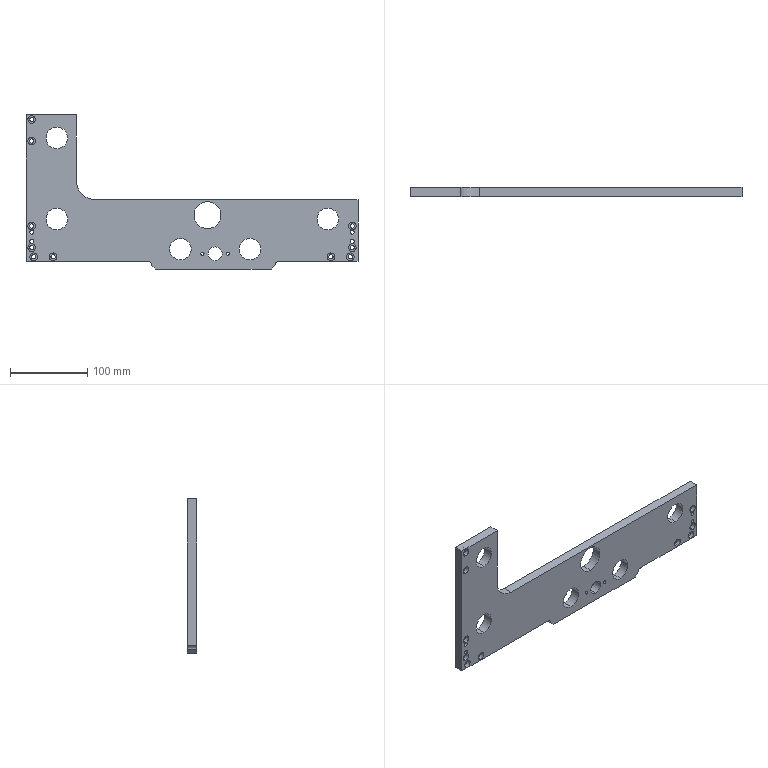Component | SolidWorks | PressingMechanism-13-1 | 1 solid | 91 faces | volume 460610 mm3 | cylinder 69 | plane 22 | commonest cylinder face diameters 10 x22 5.5 x20 28 x10 5 x8 4.2 x4 35 x2 18 x2 50 x1